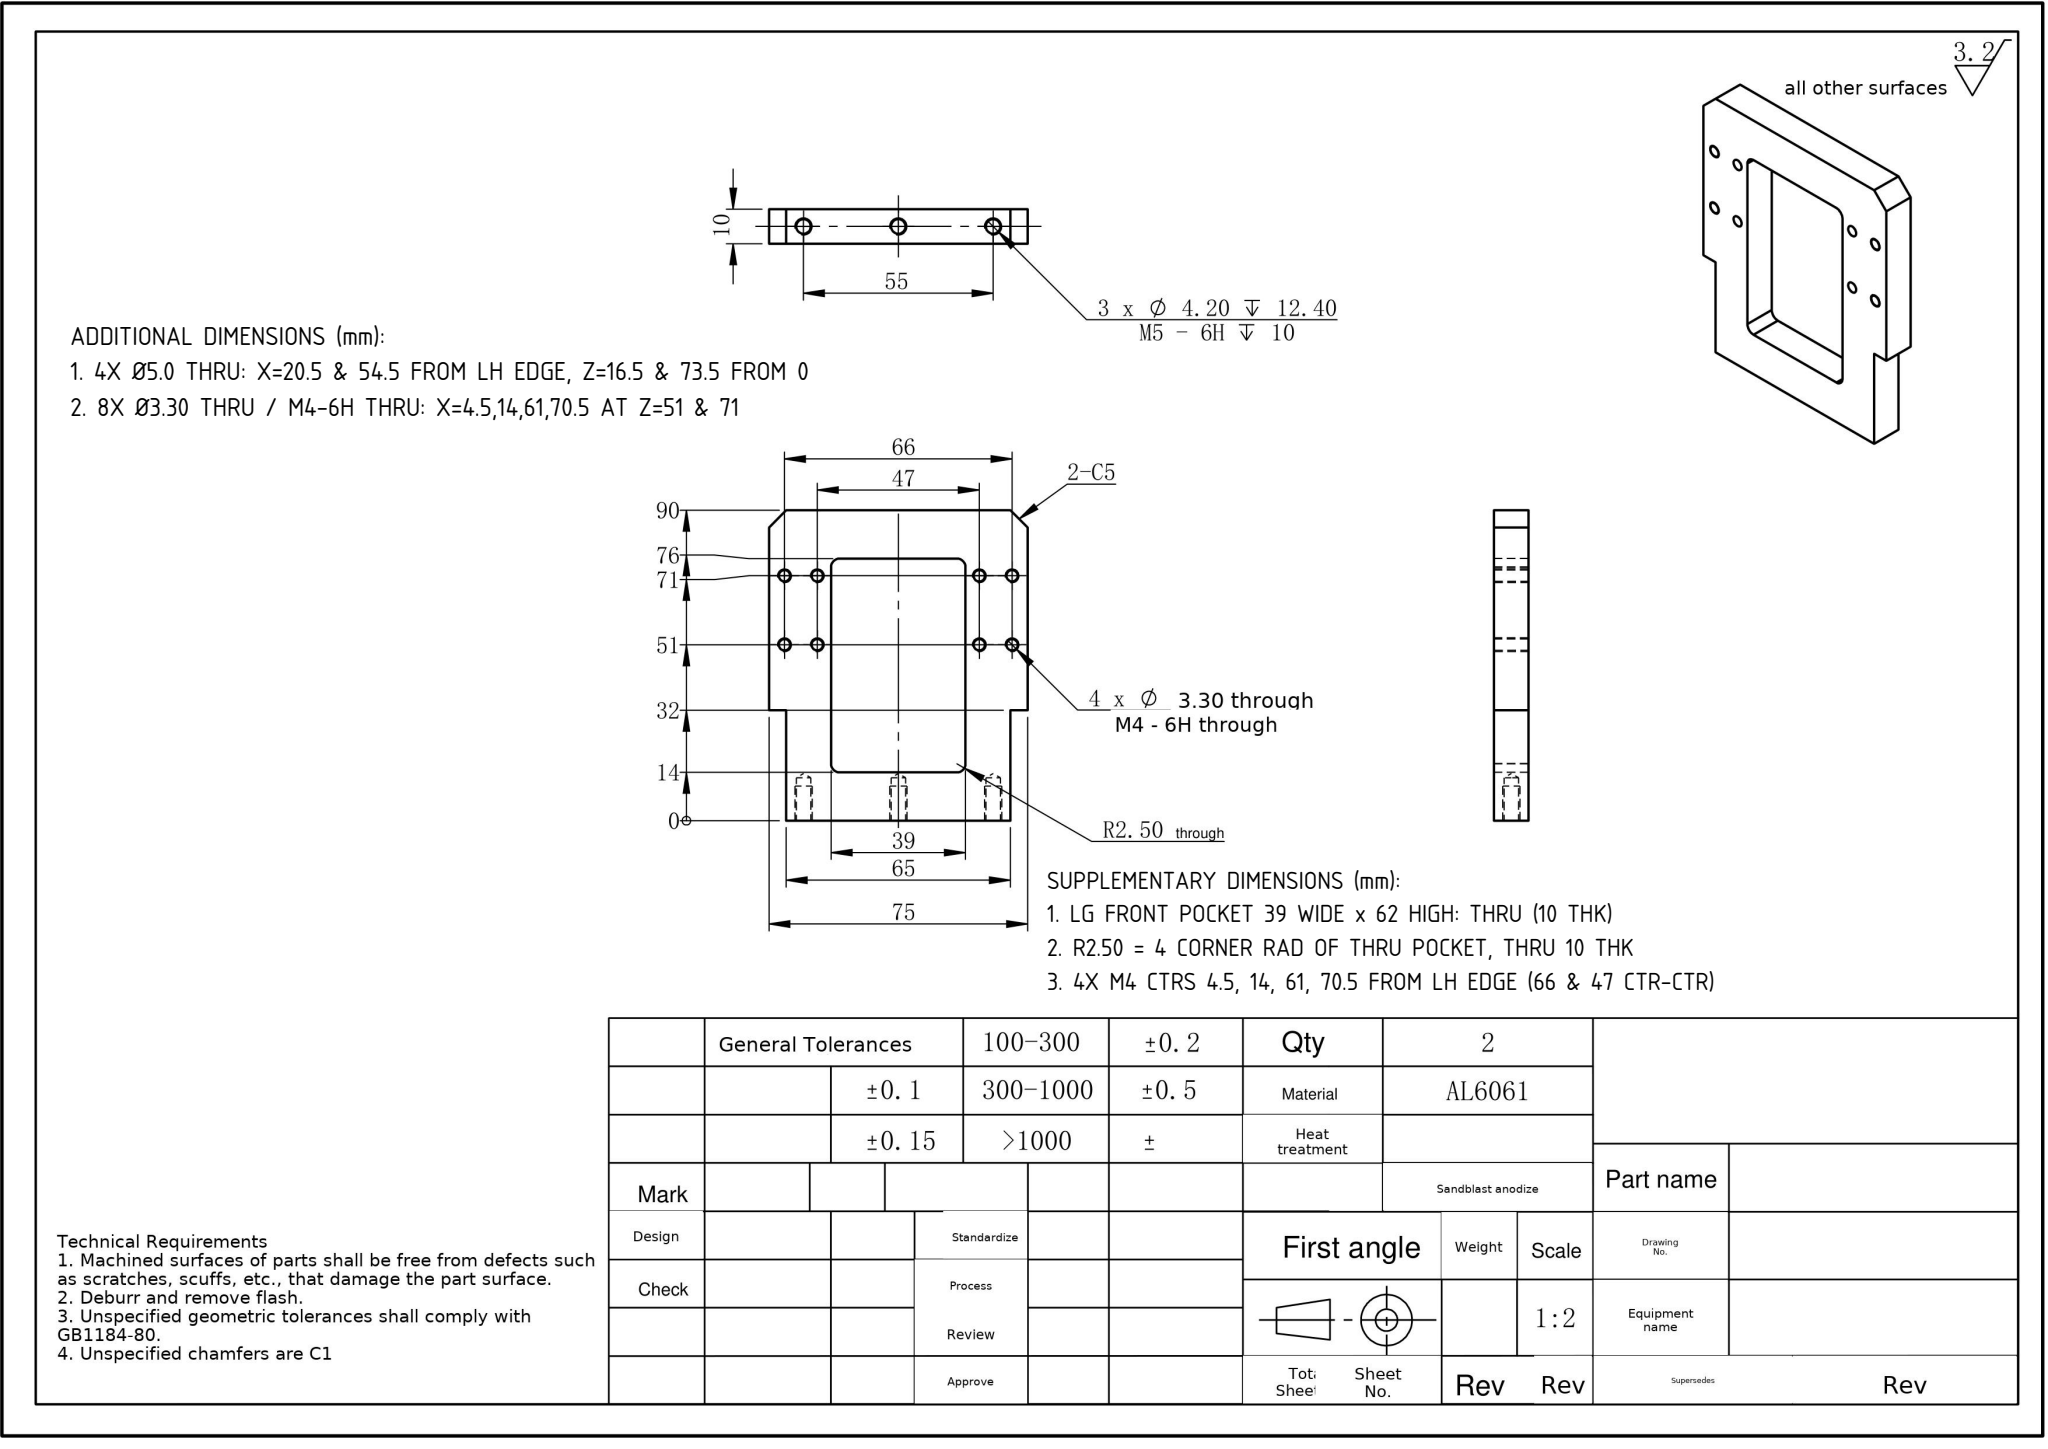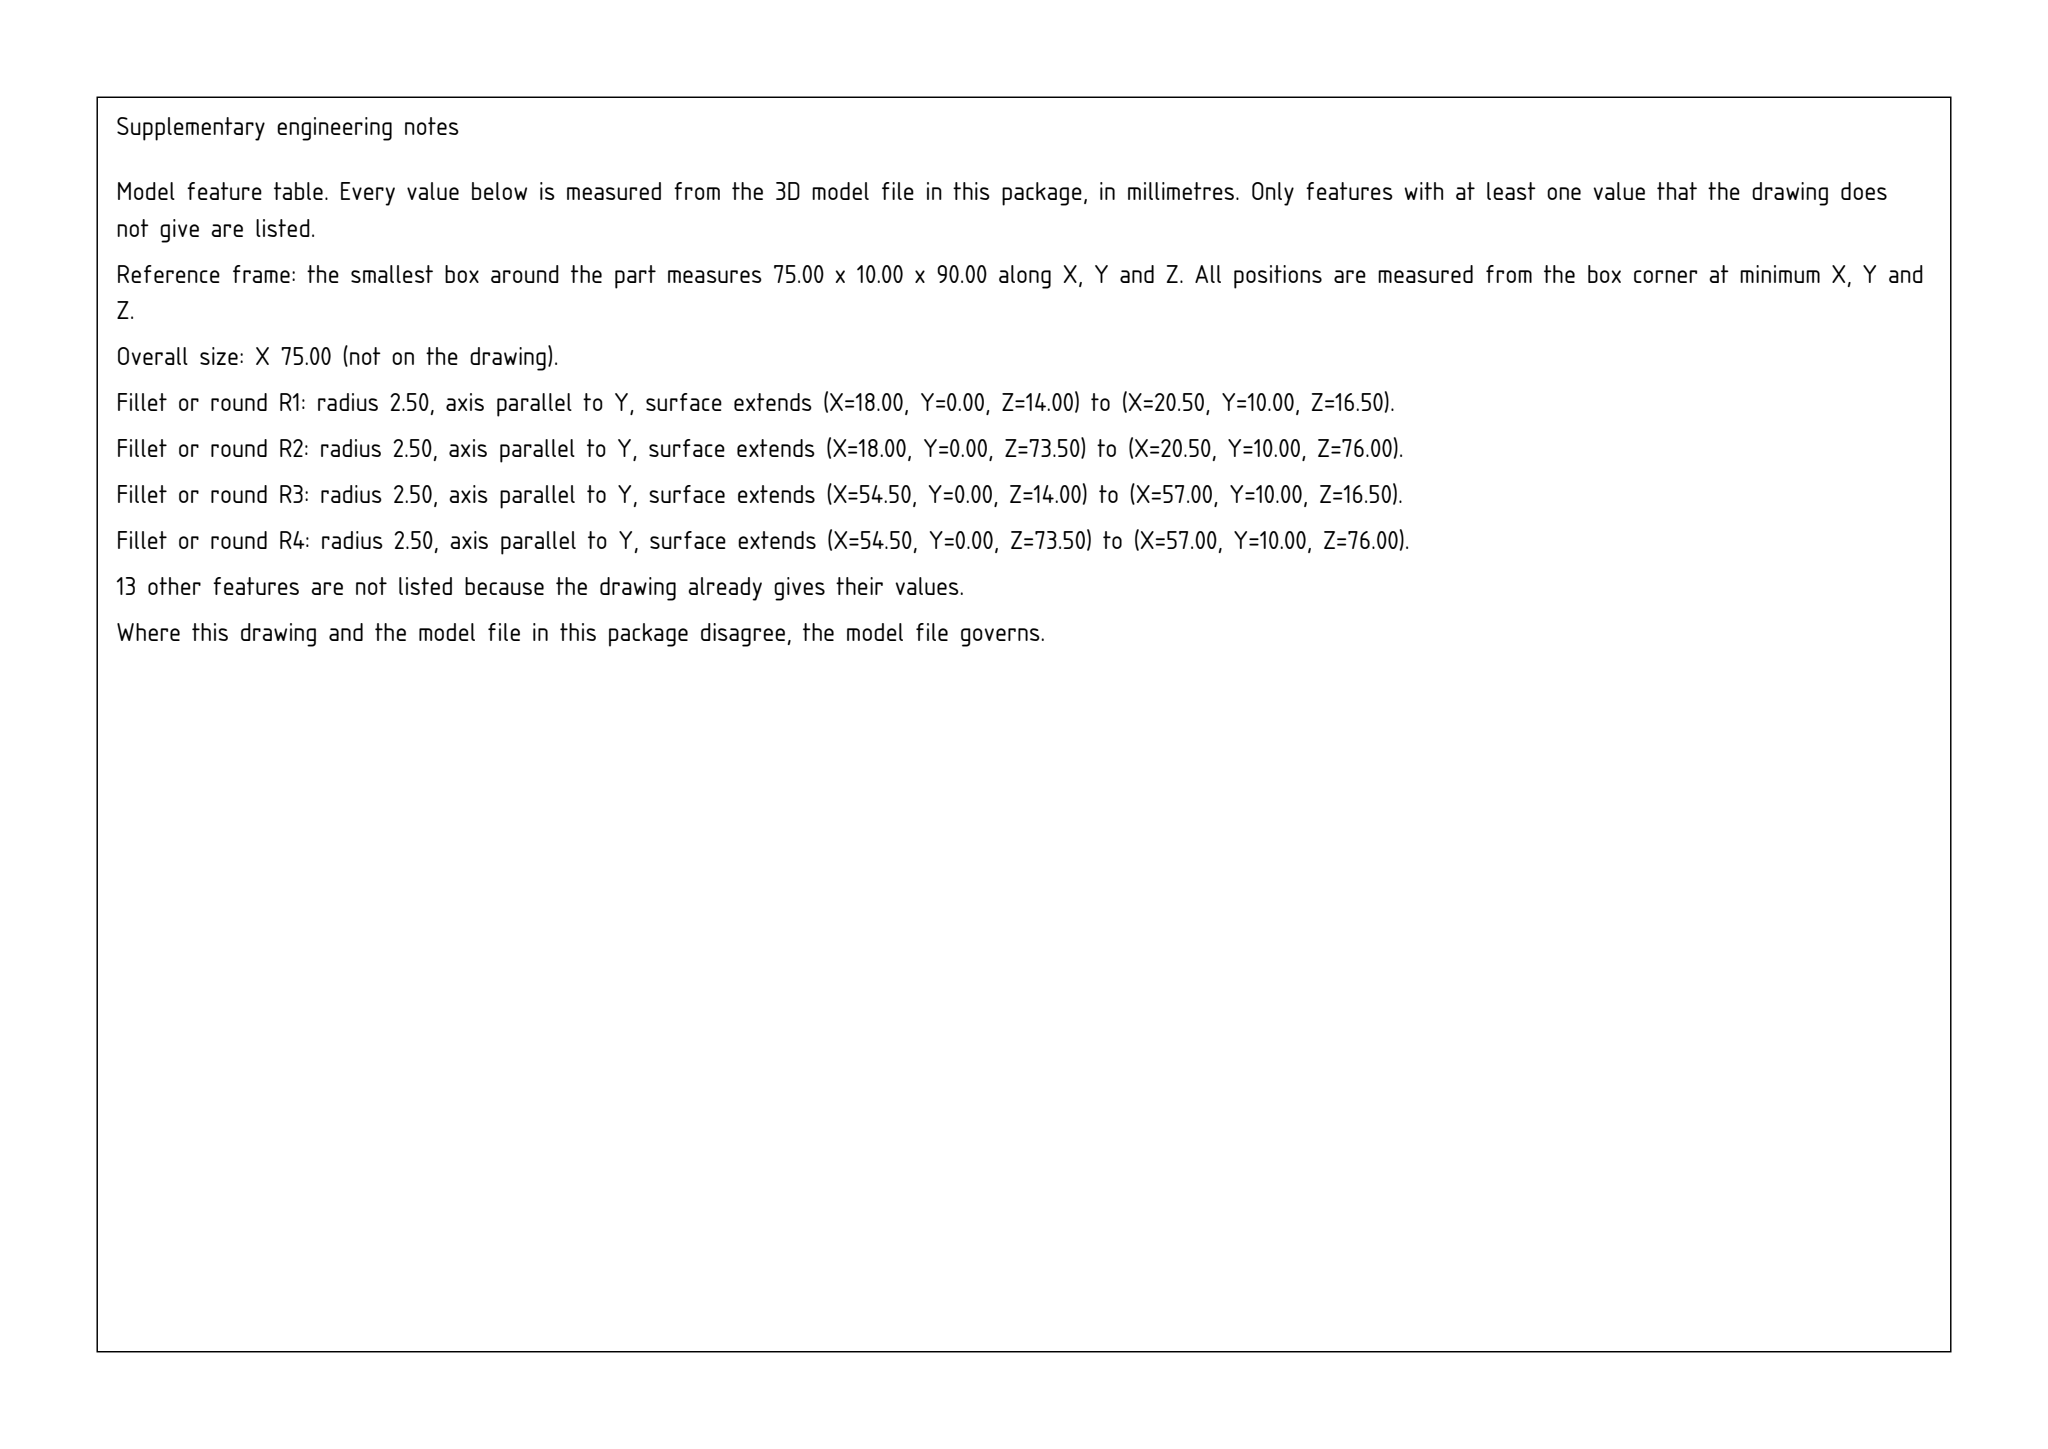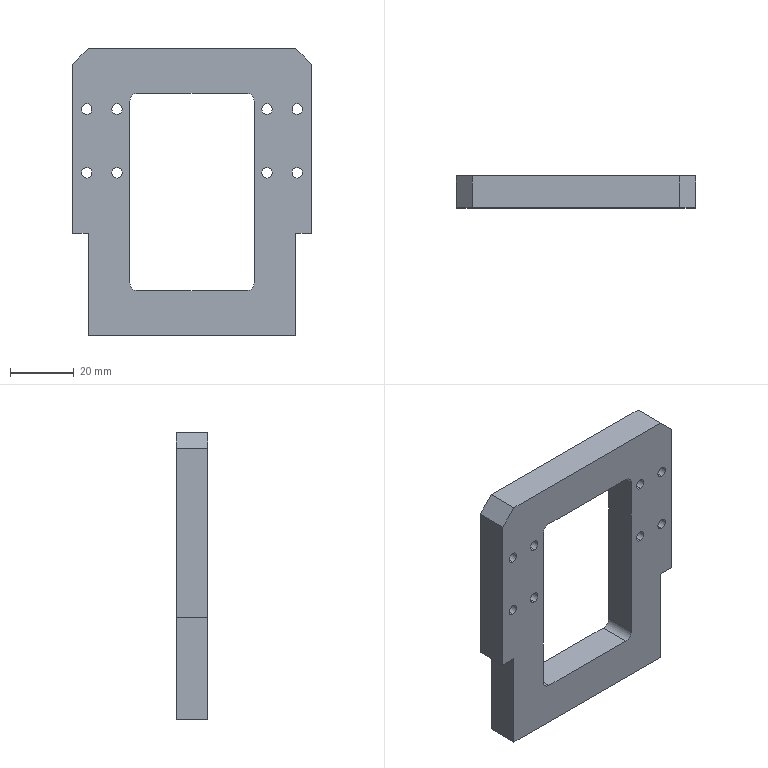Part | SolidWorks | mm | 1 solid | 48 faces | box 75 x 10 x 90 mm | volume 38707 mm3 | cylinder 26 | plane 16 | cone 6 | commonest cylinder face diameters 3.3 x16 4.2 x6 5 x4
build123d program:
from build123d import *

# Parameters (mm, degrees)
SKETCH1_W             = 75
SKETCH1_H             = 90
BOSS_EXTRUDE1_DEPTH   = 5
M5_TAPPED_HOLE1_D     = 4.2
M5_TAPPED_HOLE1_DEPTH = 12.4
M5_TAPPED_HOLE1_TIP   = 1.262
CHAMFER1_SIZE         = 5
SKETCH6_W             = 5
SKETCH6_H             = 10
CUT_EXTRUDE1_DEPTH    = 32
CUT_EXTRUDE2_DEPTH    = 30
M4_TAPPED_HOLE1_D     = 3.3
M4_TAPPED_HOLE2_D     = 3.3


with BuildPart() as part:
    # Sketch1 → Boss-Extrude1 (new, symmetric)
    with BuildSketch(Plane(origin=(0, 0, 0), x_dir=(1, 0, 0), z_dir=(0, 1, 0))):
        Rectangle(SKETCH1_W, SKETCH1_H)
    extrude(amount=BOSS_EXTRUDE1_DEPTH, both=True)

    # M5 Tapped Hole1
    with Locations(Plane(origin=(0, 0, -45), x_dir=(-1, 0, 0), z_dir=(0, 0, -1))):
        with Locations((0, 0), (-27.5, 0), (27.5, 0)):
            Hole(M5_TAPPED_HOLE1_D / 2, depth=M5_TAPPED_HOLE1_DEPTH)
            with Locations((0, 0, -(M5_TAPPED_HOLE1_DEPTH + M5_TAPPED_HOLE1_TIP / 2))):  # 118° drill point
                Cone(0, M5_TAPPED_HOLE1_D / 2, M5_TAPPED_HOLE1_TIP, mode=Mode.SUBTRACT)

    # Chamfer1
    chamfer1_edges = [part.edges().sort_by_distance(p)[0] for p in [
        (37.5, 0, 45),
        (-37.5, 0, 45),
    ]]
    chamfer(chamfer1_edges, length=CHAMFER1_SIZE)

    # Sketch6 → Cut-Extrude1 (cut)
    with BuildSketch(Plane(origin=(0, 0, -45), x_dir=(-1, 0, 0), z_dir=(0, 0, -1))):
        with Locations((35, 0)):
            Rectangle(SKETCH6_W, SKETCH6_H)
        with Locations((-35, 0)):
            Rectangle(SKETCH6_W, SKETCH6_H)
    extrude(amount=-CUT_EXTRUDE1_DEPTH, mode=Mode.SUBTRACT)

    # Sketch7 → Cut-Extrude2 (cut)
    with BuildSketch(Plane(origin=(0, 5, 0), x_dir=(1, 0, 0), z_dir=(0, 1, 0))):
        with BuildLine():
            Line((-17, 31), (17, 31))
            ThreePointArc((17, 31), (18.768, 30.268), (19.5, 28.5))
            Line((19.5, 28.5), (19.5, -28.5))
            ThreePointArc((19.5, -28.5), (18.768, -30.268), (17, -31))
            Line((17, -31), (-17, -31))
            ThreePointArc((-17, -31), (-18.768, -30.268), (-19.5, -28.5))
            Line((-19.5, -28.5), (-19.5, 28.5))
            ThreePointArc((-19.5, 28.5), (-18.768, 30.268), (-17, 31))
        make_face()
    extrude(amount=-CUT_EXTRUDE2_DEPTH, mode=Mode.SUBTRACT)

    # M4 Tapped Hole1 (through all)
    with Locations(Plane(origin=(0, -5, 0), x_dir=(-1, 0, 0), z_dir=(0, -1, 0))):
        with Locations((-33, -26), (-33, -6), (33, -26), (33, -6)):
            Hole(M4_TAPPED_HOLE1_D / 2)

    # M4 Tapped Hole2 (through all)
    with Locations(Plane(origin=(0, 5, 0), x_dir=(1, 0, 0), z_dir=(0, 1, 0))):
        with Locations((-23.5, -26), (-23.5, -6), (23.5, -6), (23.5, -26)):
            Hole(M4_TAPPED_HOLE2_D / 2)


solid = part.part